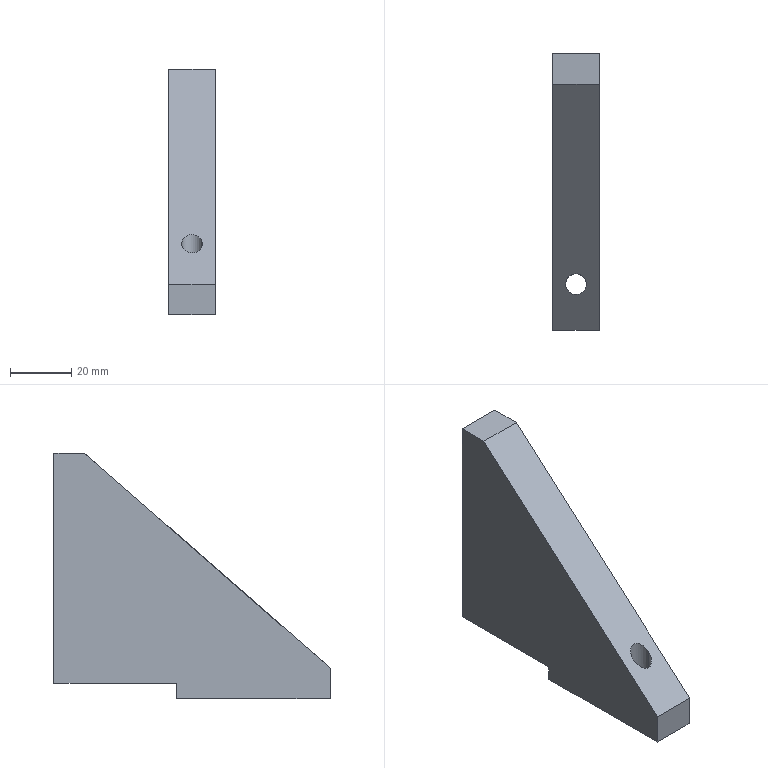Component | SolidWorks | FrameAssembly-1_SupportBlock-2 | 1 solid | 31 faces | box 15 x 90 x 80 mm | volume 59644 mm3 | cone 14 | plane 9 | cylinder 8 | commonest cylinder face diameters 6.8 x8
build123d program:
from build123d import *

# Parameters (mm, degrees)
BOSS_EXTRUDE1_DEPTH            = 15
SKETCH2_W                      = 5
SKETCH2_H                      = 40
CUT_EXTRUDE1_DEPTH             = 122.347
F_6_8_6_8_DIAMETER_HOLE1_D     = 6.8
F_6_8_6_8_DIAMETER_HOLE2_D     = 6.8
F_6_8_6_8_DIAMETER_HOLE2_DEPTH = 22.25
F_6_8_6_8_DIAMETER_HOLE2_TIP   = 2.043
F_6_8_6_8_DIAMETER_HOLE3_D     = 6.8
F_6_8_6_8_DIAMETER_HOLE3_DEPTH = 22.25
F_6_8_6_8_DIAMETER_HOLE3_TIP   = 2.043
CHAMFER1_SIZE                  = 0.625


with BuildPart() as part:
    # Sketch1 → Boss-Extrude1 (new body)
    with BuildSketch(Plane.XY.offset(7.5)):
        Polygon((80, 80), (80, 90), (0, 90), (0, 0), (10, 0), align=None)
    extrude(amount=-BOSS_EXTRUDE1_DEPTH)

    # Sketch2 → Cut-Extrude1 (cut, through all)
    with BuildSketch(Plane(origin=(0, 0, -7.5), x_dir=(-1, 0, 0), z_dir=(0, 0, -1))):
        with Locations((-2.5, 70)):
            Rectangle(SKETCH2_W, SKETCH2_H)
    extrude(amount=-CUT_EXTRUDE1_DEPTH, mode=Mode.SUBTRACT)

    # 6.8 _6.8_ Diameter Hole1 (through all)
    with Locations(Plane.ZY):
        with Locations((0, 15)):
            Hole(F_6_8_6_8_DIAMETER_HOLE1_D / 2)

    # 6.8 _6.8_ Diameter Hole2
    with Locations(Plane(origin=(0, 90, 0), x_dir=(1, 0, 0), z_dir=(0, 1, 0))):
        with Locations((60, 0), (20, 0)):
            Hole(F_6_8_6_8_DIAMETER_HOLE2_D / 2, depth=F_6_8_6_8_DIAMETER_HOLE2_DEPTH)
            with Locations((0, 0, -(F_6_8_6_8_DIAMETER_HOLE2_DEPTH + F_6_8_6_8_DIAMETER_HOLE2_TIP / 2))):  # 118° drill point
                Cone(0, F_6_8_6_8_DIAMETER_HOLE2_D / 2, F_6_8_6_8_DIAMETER_HOLE2_TIP, mode=Mode.SUBTRACT)

    # 6.8 _6.8_ Diameter Hole3
    with Locations(Plane.ZY):
        with Locations((0, 40)):
            Hole(F_6_8_6_8_DIAMETER_HOLE3_D / 2, depth=F_6_8_6_8_DIAMETER_HOLE3_DEPTH)
            with Locations((0, 0, -(F_6_8_6_8_DIAMETER_HOLE3_DEPTH + F_6_8_6_8_DIAMETER_HOLE3_TIP / 2))):  # 118° drill point
                Cone(0, F_6_8_6_8_DIAMETER_HOLE3_D / 2, F_6_8_6_8_DIAMETER_HOLE3_TIP, mode=Mode.SUBTRACT)

    # Chamfer1
    chamfer1_edges = [part.edges().sort_by_distance(p)[0] for p in [
        (0, 15, 3.4),
        (23.4, 90, 0),
        (63.4, 90, 0),
        (0, 40, 3.4),
    ]]
    chamfer(chamfer1_edges, length=CHAMFER1_SIZE)


solid = part.part

# Placed as in the assembly
solid = solid.moved(Location((-141.246, 270.373, -16.5), (0, -90, 0)))
STEP:
#1=COLOUR_RGB('',0.7922,0.8196,0.9333);
#2=FILL_AREA_STYLE_COLOUR('',#1);
#3=FILL_AREA_STYLE('',(#2));
#4=SURFACE_STYLE_FILL_AREA(#3);
#5=SURFACE_SIDE_STYLE('',(#4));
#6=SURFACE_STYLE_USAGE(.BOTH.,#5);
#7=PRESENTATION_STYLE_ASSIGNMENT((#6));
#8=CARTESIAN_POINT('',(-5.427,12.219,-0.625));
#9=VERTEX_POINT('',#8);
#10=CARTESIAN_POINT('',(-5.695,12.219,-0.625));
#11=VERTEX_POINT('',#10);
#12=CARTESIAN_POINT('',(-5.561,12.219,-0.625));
#13=DIRECTION('',(-0.,0.,-1.));
#14=DIRECTION('',(-1.,0.,0.));
#15=AXIS2_PLACEMENT_3D('',#12,#13,#14);
#16=CIRCLE('',#15,0.1339);
#17=EDGE_CURVE('',#9,#11,#16,.T.);
#18=ORIENTED_EDGE('',*,*,#17,.F.);
#19=CARTESIAN_POINT('',(-5.402,12.219,-0.6496));
#20=VERTEX_POINT('',#19);
#21=CARTESIAN_POINT('',(-5.427,12.219,-0.625));
#22=DIRECTION('',(0.7071,0.,-0.7071));
#23=VECTOR('',#22,39.37);
#24=LINE('',#21,#23);
#25=EDGE_CURVE('',#9,#20,#24,.T.);
#26=ORIENTED_EDGE('',*,*,#25,.T.);
#27=CARTESIAN_POINT('',(-5.719,12.219,-0.6496));
#28=VERTEX_POINT('',#27);
#29=CARTESIAN_POINT('',(-5.561,12.219,-0.6496));
#30=DIRECTION('',(-0.,0.,1.));
#31=DIRECTION('',(0.,-1.,0.));
#32=AXIS2_PLACEMENT_3D('',#29,#30,#31);
#33=CIRCLE('',#32,0.1585);
#34=EDGE_CURVE('',#28,#20,#33,.T.);
#35=ORIENTED_EDGE('',*,*,#34,.F.);
#36=CARTESIAN_POINT('',(-5.695,12.219,-0.625));
#37=DIRECTION('',(-0.7071,-0.,-0.7071));
#38=VECTOR('',#37,39.37);
#39=LINE('',#36,#38);
#40=EDGE_CURVE('',#11,#28,#39,.T.);
#41=ORIENTED_EDGE('',*,*,#40,.F.);
#42=EDGE_LOOP('',(#18,#26,#35,#41));
#43=FACE_OUTER_BOUND('',#42,.T.);
#44=CARTESIAN_POINT('',(-5.561,12.219,-0.625));
#45=DIRECTION('',(-0.,0.,-1.));
#46=DIRECTION('',(-1.,0.,0.));
#47=AXIS2_PLACEMENT_3D('',#44,#45,#46);
#48=CONICAL_SURFACE('',#47,0.1339,0.7854);
#49=ADVANCED_FACE('',(#43),#48,.F.);
#50=CARTESIAN_POINT('',(-5.427,11.235,-0.625));
#51=VERTEX_POINT('',#50);
#52=CARTESIAN_POINT('',(-5.695,11.235,-0.625));
#53=VERTEX_POINT('',#52);
#54=CARTESIAN_POINT('',(-5.561,11.235,-0.625));
#55=DIRECTION('',(-0.,0.,-1.));
#56=DIRECTION('',(-1.,0.,0.));
#57=AXIS2_PLACEMENT_3D('',#54,#55,#56);
#58=CIRCLE('',#57,0.1339);
#59=EDGE_CURVE('',#51,#53,#58,.T.);
#60=ORIENTED_EDGE('',*,*,#59,.F.);
#61=CARTESIAN_POINT('',(-5.402,11.235,-0.6496));
#62=VERTEX_POINT('',#61);
#63=CARTESIAN_POINT('',(-5.427,11.235,-0.625));
#64=DIRECTION('',(0.7071,0.,-0.7071));
#65=VECTOR('',#64,39.37);
#66=LINE('',#63,#65);
#67=EDGE_CURVE('',#51,#62,#66,.T.);
#68=ORIENTED_EDGE('',*,*,#67,.T.);
#69=CARTESIAN_POINT('',(-5.719,11.235,-0.6496));
#70=VERTEX_POINT('',#69);
#71=CARTESIAN_POINT('',(-5.561,11.235,-0.6496));
#72=DIRECTION('',(-0.,0.,1.));
#73=DIRECTION('',(0.,-1.,0.));
#74=AXIS2_PLACEMENT_3D('',#71,#72,#73);
#75=CIRCLE('',#74,0.1585);
#76=EDGE_CURVE('',#70,#62,#75,.T.);
#77=ORIENTED_EDGE('',*,*,#76,.F.);
#78=CARTESIAN_POINT('',(-5.695,11.235,-0.625));
#79=DIRECTION('',(-0.7071,0.,-0.7071));
#80=VECTOR('',#79,39.37);
#81=LINE('',#78,#80);
#82=EDGE_CURVE('',#53,#70,#81,.T.);
#83=ORIENTED_EDGE('',*,*,#82,.F.);
#84=EDGE_LOOP('',(#60,#68,#77,#83));
#85=FACE_OUTER_BOUND('',#84,.T.);
#86=CARTESIAN_POINT('',(-5.561,11.235,-0.625));
#87=DIRECTION('',(-0.,0.,-1.));
#88=DIRECTION('',(-1.,0.,0.));
#89=AXIS2_PLACEMENT_3D('',#86,#87,#88);
#90=CONICAL_SURFACE('',#89,0.1339,0.7854);
#91=ADVANCED_FACE('',(#85),#90,.F.);
#92=CARTESIAN_POINT('',(-5.427,14.163,1.713));
#93=VERTEX_POINT('',#92);
#94=CARTESIAN_POINT('',(-5.695,14.163,1.713));
#95=VERTEX_POINT('',#94);
#96=CARTESIAN_POINT('',(-5.561,14.163,1.713));
#97=DIRECTION('',(-0.,1.,0.));
#98=DIRECTION('',(-1.,0.,0.));
#99=AXIS2_PLACEMENT_3D('',#96,#97,#98);
#100=CIRCLE('',#99,0.1339);
#101=EDGE_CURVE('',#93,#95,#100,.T.);
#102=ORIENTED_EDGE('',*,*,#101,.F.);
#103=CARTESIAN_POINT('',(-5.402,14.188,1.713));
#104=VERTEX_POINT('',#103);
#105=CARTESIAN_POINT('',(-5.427,14.163,1.713));
#106=DIRECTION('',(0.7071,0.7071,0.));
#107=VECTOR('',#106,39.37);
#108=LINE('',#105,#107);
#109=EDGE_CURVE('',#93,#104,#108,.T.);
#110=ORIENTED_EDGE('',*,*,#109,.T.);
#111=CARTESIAN_POINT('',(-5.719,14.188,1.713));
#112=VERTEX_POINT('',#111);
#113=CARTESIAN_POINT('',(-5.561,14.188,1.713));
#114=DIRECTION('',(0.,-1.,0.));
#115=DIRECTION('',(0.,0.,-1.));
#116=AXIS2_PLACEMENT_3D('',#113,#114,#115);
#117=CIRCLE('',#116,0.1585);
#118=EDGE_CURVE('',#112,#104,#117,.T.);
#119=ORIENTED_EDGE('',*,*,#118,.F.);
#120=CARTESIAN_POINT('',(-5.695,14.163,1.713));
#121=DIRECTION('',(-0.7071,0.7071,0.));
#122=VECTOR('',#121,39.37);
#123=LINE('',#120,#122);
#124=EDGE_CURVE('',#95,#112,#123,.T.);
#125=ORIENTED_EDGE('',*,*,#124,.F.);
#126=EDGE_LOOP('',(#102,#110,#119,#125));
#127=FACE_OUTER_BOUND('',#126,.T.);
#128=CARTESIAN_POINT('',(-5.561,14.163,1.713));
#129=DIRECTION('',(-0.,1.,0.));
#130=DIRECTION('',(-1.,0.,0.));
#131=AXIS2_PLACEMENT_3D('',#128,#129,#130);
#132=CONICAL_SURFACE('',#131,0.1339,0.7854);
#133=ADVANCED_FACE('',(#127),#132,.F.);
#134=CARTESIAN_POINT('',(-5.427,14.163,0.1378));
#135=VERTEX_POINT('',#134);
#136=CARTESIAN_POINT('',(-5.695,14.163,0.1378));
#137=VERTEX_POINT('',#136);
#138=CARTESIAN_POINT('',(-5.561,14.163,0.1378));
#139=DIRECTION('',(-0.,1.,0.));
#140=DIRECTION('',(-1.,0.,0.));
#141=AXIS2_PLACEMENT_3D('',#138,#139,#140);
#142=CIRCLE('',#141,0.1339);
#143=EDGE_CURVE('',#135,#137,#142,.T.);
#144=ORIENTED_EDGE('',*,*,#143,.F.);
#145=CARTESIAN_POINT('',(-5.402,14.188,0.1378));
#146=VERTEX_POINT('',#145);
#147=CARTESIAN_POINT('',(-5.427,14.163,0.1378));
#148=DIRECTION('',(0.7071,0.7071,0.));
#149=VECTOR('',#148,39.37);
#150=LINE('',#147,#149);
#151=EDGE_CURVE('',#135,#146,#150,.T.);
#152=ORIENTED_EDGE('',*,*,#151,.T.);
#153=CARTESIAN_POINT('',(-5.719,14.188,0.1378));
#154=VERTEX_POINT('',#153);
#155=CARTESIAN_POINT('',(-5.561,14.188,0.1378));
#156=DIRECTION('',(0.,-1.,0.));
#157=DIRECTION('',(0.,0.,-1.));
#158=AXIS2_PLACEMENT_3D('',#155,#156,#157);
#159=CIRCLE('',#158,0.1585);
#160=EDGE_CURVE('',#154,#146,#159,.T.);
#161=ORIENTED_EDGE('',*,*,#160,.F.);
#162=CARTESIAN_POINT('',(-5.695,14.163,0.1378));
#163=DIRECTION('',(-0.7071,0.7071,0.));
#164=VECTOR('',#163,39.37);
#165=LINE('',#162,#164);
#166=EDGE_CURVE('',#137,#154,#165,.T.);
#167=ORIENTED_EDGE('',*,*,#166,.F.);
#168=EDGE_LOOP('',(#144,#152,#161,#167));
#169=FACE_OUTER_BOUND('',#168,.T.);
#170=CARTESIAN_POINT('',(-5.561,14.163,0.1378));
#171=DIRECTION('',(-0.,1.,0.));
#172=DIRECTION('',(-1.,0.,0.));
#173=AXIS2_PLACEMENT_3D('',#170,#171,#172);
#174=CONICAL_SURFACE('',#173,0.1339,0.7854);
#175=ADVANCED_FACE('',(#169),#174,.F.);
#176=CARTESIAN_POINT('',(-5.427,12.219,0.2264));
#177=VERTEX_POINT('',#176);
#178=CARTESIAN_POINT('',(-5.695,12.219,0.2264));
#179=VERTEX_POINT('',#178);
#180=CARTESIAN_POINT('',(-5.561,12.219,0.2264));
#181=DIRECTION('',(-0.,0.,-1.));
#182=DIRECTION('',(-1.,0.,0.));
#183=AXIS2_PLACEMENT_3D('',#180,#181,#182);
#184=CIRCLE('',#183,0.1339);
#185=EDGE_CURVE('',#177,#179,#184,.T.);
#186=ORIENTED_EDGE('',*,*,#185,.F.);
#187=CARTESIAN_POINT('',(-5.427,12.219,-0.6496));
#188=DIRECTION('',(-0.,0.,-1.));
#189=VECTOR('',#188,39.37);
#190=LINE('',#187,#189);
#191=EDGE_CURVE('',#177,#9,#190,.T.);
#192=ORIENTED_EDGE('',*,*,#191,.T.);
#193=ORIENTED_EDGE('',*,*,#17,.T.);
#194=CARTESIAN_POINT('',(-5.695,12.219,-0.6496));
#195=DIRECTION('',(-0.,0.,-1.));
#196=VECTOR('',#195,39.37);
#197=LINE('',#194,#196);
#198=EDGE_CURVE('',#179,#11,#197,.T.);
#199=ORIENTED_EDGE('',*,*,#198,.F.);
#200=EDGE_LOOP('',(#186,#192,#193,#199));
#201=FACE_OUTER_BOUND('',#200,.T.);
#202=CARTESIAN_POINT('',(-5.561,12.219,-0.6496));
#203=DIRECTION('',(-0.,0.,-1.));
#204=DIRECTION('',(-1.,0.,0.));
#205=AXIS2_PLACEMENT_3D('',#202,#203,#204);
#206=CYLINDRICAL_SURFACE('',#205,0.1339);
#207=ADVANCED_FACE('',(#201),#206,.F.);
#208=CARTESIAN_POINT('',(-5.561,12.219,0.3068));
#209=VERTEX_POINT('',#208);
#210=CARTESIAN_POINT('',(-5.695,12.219,0.2264));
#211=DIRECTION('',(-0.8572,-0.,-0.515));
#212=VECTOR('',#211,39.37);
#213=LINE('',#210,#212);
#214=EDGE_CURVE('',#209,#179,#213,.T.);
#215=ORIENTED_EDGE('',*,*,#214,.F.);
#216=CARTESIAN_POINT('',(-5.427,12.219,0.2264));
#217=DIRECTION('',(0.8572,0.,-0.515));
#218=VECTOR('',#217,39.37);
#219=LINE('',#216,#218);
#220=EDGE_CURVE('',#209,#177,#219,.T.);
#221=ORIENTED_EDGE('',*,*,#220,.T.);
#222=ORIENTED_EDGE('',*,*,#185,.T.);
#223=EDGE_LOOP('',(#215,#221,#222));
#224=FACE_OUTER_BOUND('',#223,.T.);
#225=CARTESIAN_POINT('',(-5.561,12.219,0.2264));
#226=DIRECTION('',(-0.,0.,-1.));
#227=DIRECTION('',(-1.,0.,0.));
#228=AXIS2_PLACEMENT_3D('',#225,#226,#227);
#229=CONICAL_SURFACE('',#228,0.1339,1.03);
#230=ADVANCED_FACE('',(#224),#229,.F.);
#231=CARTESIAN_POINT('',(-5.427,13.312,1.713));
#232=VERTEX_POINT('',#231);
#233=CARTESIAN_POINT('',(-5.695,13.312,1.713));
#234=VERTEX_POINT('',#233);
#235=CARTESIAN_POINT('',(-5.561,13.312,1.713));
#236=DIRECTION('',(-0.,1.,0.));
#237=DIRECTION('',(-1.,0.,0.));
#238=AXIS2_PLACEMENT_3D('',#235,#236,#237);
#239=CIRCLE('',#238,0.1339);
#240=EDGE_CURVE('',#232,#234,#239,.T.);
#241=ORIENTED_EDGE('',*,*,#240,.F.);
#242=CARTESIAN_POINT('',(-5.427,14.188,1.713));
#243=DIRECTION('',(-0.,1.,0.));
#244=VECTOR('',#243,39.37);
#245=LINE('',#242,#244);
#246=EDGE_CURVE('',#232,#93,#245,.T.);
#247=ORIENTED_EDGE('',*,*,#246,.T.);
#248=ORIENTED_EDGE('',*,*,#101,.T.);
#249=CARTESIAN_POINT('',(-5.695,14.188,1.713));
#250=DIRECTION('',(-0.,1.,0.));
#251=VECTOR('',#250,39.37);
#252=LINE('',#249,#251);
#253=EDGE_CURVE('',#234,#95,#252,.T.);
#254=ORIENTED_EDGE('',*,*,#253,.F.);
#255=EDGE_LOOP('',(#241,#247,#248,#254));
#256=FACE_OUTER_BOUND('',#255,.T.);
#257=CARTESIAN_POINT('',(-5.561,14.188,1.713));
#258=DIRECTION('',(-0.,1.,0.));
#259=DIRECTION('',(-1.,0.,0.));
#260=AXIS2_PLACEMENT_3D('',#257,#258,#259);
#261=CYLINDRICAL_SURFACE('',#260,0.1339);
#262=ADVANCED_FACE('',(#256),#261,.F.);
#263=CARTESIAN_POINT('',(-5.561,13.232,1.713));
#264=VERTEX_POINT('',#263);
#265=CARTESIAN_POINT('',(-5.695,13.312,1.713));
#266=DIRECTION('',(-0.8572,0.515,0.));
#267=VECTOR('',#266,39.37);
#268=LINE('',#265,#267);
#269=EDGE_CURVE('',#264,#234,#268,.T.);
#270=ORIENTED_EDGE('',*,*,#269,.F.);
#271=CARTESIAN_POINT('',(-5.427,13.312,1.713));
#272=DIRECTION('',(0.8572,0.515,0.));
#273=VECTOR('',#272,39.37);
#274=LINE('',#271,#273);
#275=EDGE_CURVE('',#264,#232,#274,.T.);
#276=ORIENTED_EDGE('',*,*,#275,.T.);
#277=ORIENTED_EDGE('',*,*,#240,.T.);
#278=EDGE_LOOP('',(#270,#276,#277));
#279=FACE_OUTER_BOUND('',#278,.T.);
#280=CARTESIAN_POINT('',(-5.561,13.312,1.713));
#281=DIRECTION('',(-0.,1.,0.));
#282=DIRECTION('',(-1.,0.,0.));
#283=AXIS2_PLACEMENT_3D('',#280,#281,#282);
#284=CONICAL_SURFACE('',#283,0.1339,1.03);
#285=ADVANCED_FACE('',(#279),#284,.F.);
#286=CARTESIAN_POINT('',(-5.427,13.312,0.1378));
#287=VERTEX_POINT('',#286);
#288=CARTESIAN_POINT('',(-5.695,13.312,0.1378));
#289=VERTEX_POINT('',#288);
#290=CARTESIAN_POINT('',(-5.561,13.312,0.1378));
#291=DIRECTION('',(-0.,1.,0.));
#292=DIRECTION('',(-1.,0.,0.));
#293=AXIS2_PLACEMENT_3D('',#290,#291,#292);
#294=CIRCLE('',#293,0.1339);
#295=EDGE_CURVE('',#287,#289,#294,.T.);
#296=ORIENTED_EDGE('',*,*,#295,.F.);
#297=CARTESIAN_POINT('',(-5.427,14.188,0.1378));
#298=DIRECTION('',(-0.,1.,0.));
#299=VECTOR('',#298,39.37);
#300=LINE('',#297,#299);
#301=EDGE_CURVE('',#287,#135,#300,.T.);
#302=ORIENTED_EDGE('',*,*,#301,.T.);
#303=ORIENTED_EDGE('',*,*,#143,.T.);
#304=CARTESIAN_POINT('',(-5.695,14.188,0.1378));
#305=DIRECTION('',(-0.,1.,0.));
#306=VECTOR('',#305,39.37);
#307=LINE('',#304,#306);
#308=EDGE_CURVE('',#289,#137,#307,.T.);
#309=ORIENTED_EDGE('',*,*,#308,.F.);
#310=EDGE_LOOP('',(#296,#302,#303,#309));
#311=FACE_OUTER_BOUND('',#310,.T.);
#312=CARTESIAN_POINT('',(-5.561,14.188,0.1378));
#313=DIRECTION('',(-0.,1.,0.));
#314=DIRECTION('',(-1.,0.,0.));
#315=AXIS2_PLACEMENT_3D('',#312,#313,#314);
#316=CYLINDRICAL_SURFACE('',#315,0.1339);
#317=ADVANCED_FACE('',(#311),#316,.F.);
#318=CARTESIAN_POINT('',(-5.561,13.232,0.1378));
#319=VERTEX_POINT('',#318);
#320=CARTESIAN_POINT('',(-5.695,13.312,0.1378));
#321=DIRECTION('',(-0.8572,0.515,0.));
#322=VECTOR('',#321,39.37);
#323=LINE('',#320,#322);
#324=EDGE_CURVE('',#319,#289,#323,.T.);
#325=ORIENTED_EDGE('',*,*,#324,.F.);
#326=CARTESIAN_POINT('',(-5.427,13.312,0.1378));
#327=DIRECTION('',(0.8572,0.515,0.));
#328=VECTOR('',#327,39.37);
#329=LINE('',#326,#328);
#330=EDGE_CURVE('',#319,#287,#329,.T.);
#331=ORIENTED_EDGE('',*,*,#330,.T.);
#332=ORIENTED_EDGE('',*,*,#295,.T.);
#333=EDGE_LOOP('',(#325,#331,#332));
#334=FACE_OUTER_BOUND('',#333,.T.);
#335=CARTESIAN_POINT('',(-5.561,13.312,0.1378));
#336=DIRECTION('',(-0.,1.,0.));
#337=DIRECTION('',(-1.,0.,0.));
#338=AXIS2_PLACEMENT_3D('',#335,#336,#337);
#339=CONICAL_SURFACE('',#338,0.1339,1.03);
#340=ADVANCED_FACE('',(#334),#339,.F.);
#341=CARTESIAN_POINT('',(-5.695,11.235,0.2608));
#342=VERTEX_POINT('',#341);
#343=CARTESIAN_POINT('',(-5.427,11.235,0.2608));
#344=VERTEX_POINT('',#343);
#345=CARTESIAN_POINT('',(-5.695,11.235,0.2608));
#346=CARTESIAN_POINT('',(-5.695,10.967,0.02657));
#347=CARTESIAN_POINT('',(-5.427,10.967,0.02657));
#348=CARTESIAN_POINT('',(-5.427,11.235,0.2608));
#349=(BOUNDED_CURVE()B_SPLINE_CURVE(3,(#345,#346,#347,#348),.UNSPECIFIED.,.F.,.F.)B_SPLINE_CURVE_WITH_KNOTS((4,4),(4.712,7.854),.UNSPECIFIED.)CURVE()GEOMETRIC_REPRESENTATION_ITEM()RATIONAL_B_SPLINE_CURVE((1.,0.3333,0.3333,1.))REPRESENTATION_ITEM(''));
#350=EDGE_CURVE('',#342,#344,#349,.T.);
#351=ORIENTED_EDGE('',*,*,#350,.T.);
#352=CARTESIAN_POINT('',(-5.427,11.235,-0.6496));
#353=DIRECTION('',(-0.,0.,-1.));
#354=VECTOR('',#353,39.37);
#355=LINE('',#352,#354);
#356=EDGE_CURVE('',#344,#51,#355,.T.);
#357=ORIENTED_EDGE('',*,*,#356,.T.);
#358=ORIENTED_EDGE('',*,*,#59,.T.);
#359=CARTESIAN_POINT('',(-5.695,11.235,-0.6496));
#360=DIRECTION('',(-0.,0.,-1.));
#361=VECTOR('',#360,39.37);
#362=LINE('',#359,#361);
#363=EDGE_CURVE('',#342,#53,#362,.T.);
#364=ORIENTED_EDGE('',*,*,#363,.F.);
#365=EDGE_LOOP('',(#351,#357,#358,#364));
#366=FACE_OUTER_BOUND('',#365,.T.);
#367=CARTESIAN_POINT('',(-5.561,11.235,-0.6496));
#368=DIRECTION('',(-0.,0.,-1.));
#369=DIRECTION('',(-1.,0.,0.));
#370=AXIS2_PLACEMENT_3D('',#367,#368,#369);
#371=CYLINDRICAL_SURFACE('',#370,0.1339);
#372=ADVANCED_FACE('',(#366),#371,.F.);
#373=ORIENTED_EDGE('',*,*,#350,.F.);
#374=CARTESIAN_POINT('',(-5.427,11.235,0.2608));
#375=CARTESIAN_POINT('',(-5.427,11.503,0.4951));
#376=CARTESIAN_POINT('',(-5.695,11.503,0.4951));
#377=CARTESIAN_POINT('',(-5.695,11.235,0.2608));
#378=(BOUNDED_CURVE()B_SPLINE_CURVE(3,(#374,#375,#376,#377),.UNSPECIFIED.,.F.,.F.)B_SPLINE_CURVE_WITH_KNOTS((4,4),(1.571,4.712),.UNSPECIFIED.)CURVE()GEOMETRIC_REPRESENTATION_ITEM()RATIONAL_B_SPLINE_CURVE((1.,0.3333,0.3333,1.))REPRESENTATION_ITEM(''));
#379=EDGE_CURVE('',#344,#342,#378,.T.);
#380=ORIENTED_EDGE('',*,*,#379,.F.);
#381=EDGE_LOOP('',(#373,#380));
#382=FACE_BOUND('',#381,.T.);
#383=CARTESIAN_POINT('',(-5.856,10.645,-0.2559));
#384=VERTEX_POINT('',#383);
#385=CARTESIAN_POINT('',(-5.856,13.794,2.5));
#386=VERTEX_POINT('',#385);
#387=CARTESIAN_POINT('',(-5.856,10.645,-0.2559));
#388=DIRECTION('',(-0.,0.7526,0.6585));
#389=VECTOR('',#388,39.37);
#390=LINE('',#387,#389);
#391=EDGE_CURVE('',#384,#386,#390,.T.);
#392=ORIENTED_EDGE('',*,*,#391,.F.);
#393=CARTESIAN_POINT('',(-5.266,10.645,-0.2559));
#394=VERTEX_POINT('',#393);
#395=CARTESIAN_POINT('',(-5.266,10.645,-0.2559));
#396=DIRECTION('',(-1.,-0.,0.));
#397=VECTOR('',#396,39.37);
#398=LINE('',#395,#397);
#399=EDGE_CURVE('',#394,#384,#398,.T.);
#400=ORIENTED_EDGE('',*,*,#399,.F.);
#401=CARTESIAN_POINT('',(-5.266,13.794,2.5));
#402=VERTEX_POINT('',#401);
#403=CARTESIAN_POINT('',(-5.266,10.645,-0.2559));
#404=DIRECTION('',(-0.,0.7526,0.6585));
#405=VECTOR('',#404,39.37);
#406=LINE('',#403,#405);
#407=EDGE_CURVE('',#394,#402,#406,.T.);
#408=ORIENTED_EDGE('',*,*,#407,.T.);
#409=CARTESIAN_POINT('',(-5.266,13.794,2.5));
#410=DIRECTION('',(-1.,-0.,0.));
#411=VECTOR('',#410,39.37);
#412=LINE('',#409,#411);
#413=EDGE_CURVE('',#402,#386,#412,.T.);
#414=ORIENTED_EDGE('',*,*,#413,.T.);
#415=EDGE_LOOP('',(#392,#400,#408,#414));
#416=FACE_OUTER_BOUND('',#415,.T.);
#417=CARTESIAN_POINT('',(-5.266,10.645,-0.2559));
#418=DIRECTION('',(0.,-0.6585,0.7526));
#419=DIRECTION('',(-0.,0.7526,0.6585));
#420=AXIS2_PLACEMENT_3D('',#417,#418,#419);
#421=PLANE('',#420);
#422=ADVANCED_FACE('',(#382,#416),#421,.T.);
#423=CARTESIAN_POINT('',(-5.856,10.645,-0.6496));
#424=VERTEX_POINT('',#423);
#425=CARTESIAN_POINT('',(-5.856,10.645,-0.6496));
#426=DIRECTION('',(-0.,0.,1.));
#427=VECTOR('',#426,39.37);
#428=LINE('',#425,#427);
#429=EDGE_CURVE('',#424,#384,#428,.T.);
#430=ORIENTED_EDGE('',*,*,#429,.F.);
#431=CARTESIAN_POINT('',(-5.266,10.645,-0.6496));
#432=VERTEX_POINT('',#431);
#433=CARTESIAN_POINT('',(-5.266,10.645,-0.6496));
#434=DIRECTION('',(-1.,-0.,0.));
#435=VECTOR('',#434,39.37);
#436=LINE('',#433,#435);
#437=EDGE_CURVE('',#432,#424,#436,.T.);
#438=ORIENTED_EDGE('',*,*,#437,.F.);
#439=CARTESIAN_POINT('',(-5.266,10.645,-0.6496));
#440=DIRECTION('',(-0.,0.,1.));
#441=VECTOR('',#440,39.37);
#442=LINE('',#439,#441);
#443=EDGE_CURVE('',#432,#394,#442,.T.);
#444=ORIENTED_EDGE('',*,*,#443,.T.);
#445=ORIENTED_EDGE('',*,*,#399,.T.);
#446=EDGE_LOOP('',(#430,#438,#444,#445));
#447=FACE_OUTER_BOUND('',#446,.T.);
#448=CARTESIAN_POINT('',(-5.266,10.645,-0.6496));
#449=DIRECTION('',(0.,-1.,0.));
#450=DIRECTION('',(-0.,0.,1.));
#451=AXIS2_PLACEMENT_3D('',#448,#449,#450);
#452=PLANE('',#451);
#453=ADVANCED_FACE('',(#447),#452,.T.);
#454=ORIENTED_EDGE('',*,*,#76,.T.);
#455=CARTESIAN_POINT('',(-5.561,11.235,-0.6496));
#456=DIRECTION('',(-0.,0.,1.));
#457=DIRECTION('',(0.,-1.,0.));
#458=AXIS2_PLACEMENT_3D('',#455,#456,#457);
#459=CIRCLE('',#458,0.1585);
#460=EDGE_CURVE('',#62,#70,#459,.T.);
#461=ORIENTED_EDGE('',*,*,#460,.T.);
#462=EDGE_LOOP('',(#454,#461));
#463=FACE_BOUND('',#462,.T.);
#464=ORIENTED_EDGE('',*,*,#34,.T.);
#465=CARTESIAN_POINT('',(-5.561,12.219,-0.6496));
#466=DIRECTION('',(-0.,0.,1.));
#467=DIRECTION('',(0.,-1.,0.));
#468=AXIS2_PLACEMENT_3D('',#465,#466,#467);
#469=CIRCLE('',#468,0.1585);
#470=EDGE_CURVE('',#20,#28,#469,.T.);
#471=ORIENTED_EDGE('',*,*,#470,.T.);
#472=EDGE_LOOP('',(#464,#471));
#473=FACE_BOUND('',#472,.T.);
#474=CARTESIAN_POINT('',(-5.856,12.613,-0.6496));
#475=VERTEX_POINT('',#474);
#476=CARTESIAN_POINT('',(-5.266,12.613,-0.6496));
#477=VERTEX_POINT('',#476);
#478=CARTESIAN_POINT('',(-5.856,12.613,-0.6496));
#479=DIRECTION('',(1.,0.,-0.));
#480=VECTOR('',#479,39.37);
#481=LINE('',#478,#480);
#482=EDGE_CURVE('',#475,#477,#481,.T.);
#483=ORIENTED_EDGE('',*,*,#482,.T.);
#484=CARTESIAN_POINT('',(-5.266,14.188,-0.6496));
#485=DIRECTION('',(0.,-1.,0.));
#486=VECTOR('',#485,39.37);
#487=LINE('',#484,#486);
#488=EDGE_CURVE('',#477,#432,#487,.T.);
#489=ORIENTED_EDGE('',*,*,#488,.T.);
#490=ORIENTED_EDGE('',*,*,#437,.T.);
#491=CARTESIAN_POINT('',(-5.856,14.188,-0.6496));
#492=DIRECTION('',(0.,-1.,0.));
#493=VECTOR('',#492,39.37);
#494=LINE('',#491,#493);
#495=EDGE_CURVE('',#475,#424,#494,.T.);
#496=ORIENTED_EDGE('',*,*,#495,.F.);
#497=EDGE_LOOP('',(#483,#489,#490,#496));
#498=FACE_OUTER_BOUND('',#497,.T.);
#499=CARTESIAN_POINT('',(-5.266,14.188,-0.6496));
#500=DIRECTION('',(0.,-0.,-1.));
#501=DIRECTION('',(0.,-1.,0.));
#502=AXIS2_PLACEMENT_3D('',#499,#500,#501);
#503=PLANE('',#502);
#504=ADVANCED_FACE('',(#463,#473,#498),#503,.T.);
#505=ORIENTED_EDGE('',*,*,#160,.T.);
#506=CARTESIAN_POINT('',(-5.561,14.188,0.1378));
#507=DIRECTION('',(0.,-1.,0.));
#508=DIRECTION('',(0.,0.,-1.));
#509=AXIS2_PLACEMENT_3D('',#506,#507,#508);
#510=CIRCLE('',#509,0.1585);
#511=EDGE_CURVE('',#146,#154,#510,.T.);
#512=ORIENTED_EDGE('',*,*,#511,.T.);
#513=EDGE_LOOP('',(#505,#512));
#514=FACE_BOUND('',#513,.T.);
#515=ORIENTED_EDGE('',*,*,#118,.T.);
#516=CARTESIAN_POINT('',(-5.561,14.188,1.713));
#517=DIRECTION('',(0.,-1.,0.));
#518=DIRECTION('',(0.,0.,-1.));
#519=AXIS2_PLACEMENT_3D('',#516,#517,#518);
#520=CIRCLE('',#519,0.1585);
#521=EDGE_CURVE('',#104,#112,#520,.T.);
#522=ORIENTED_EDGE('',*,*,#521,.T.);
#523=EDGE_LOOP('',(#515,#522));
#524=FACE_BOUND('',#523,.T.);
#525=CARTESIAN_POINT('',(-5.856,14.188,-0.4528));
#526=VERTEX_POINT('',#525);
#527=CARTESIAN_POINT('',(-5.266,14.188,-0.4528));
#528=VERTEX_POINT('',#527);
#529=CARTESIAN_POINT('',(-5.856,14.188,-0.4528));
#530=DIRECTION('',(1.,0.,-0.));
#531=VECTOR('',#530,39.37);
#532=LINE('',#529,#531);
#533=EDGE_CURVE('',#526,#528,#532,.T.);
#534=ORIENTED_EDGE('',*,*,#533,.F.);
#535=CARTESIAN_POINT('',(-5.856,14.188,2.5));
#536=VERTEX_POINT('',#535);
#537=CARTESIAN_POINT('',(-5.856,14.188,2.5));
#538=DIRECTION('',(0.,-0.,-1.));
#539=VECTOR('',#538,39.37);
#540=LINE('',#537,#539);
#541=EDGE_CURVE('',#536,#526,#540,.T.);
#542=ORIENTED_EDGE('',*,*,#541,.F.);
#543=CARTESIAN_POINT('',(-5.266,14.188,2.5));
#544=VERTEX_POINT('',#543);
#545=CARTESIAN_POINT('',(-5.266,14.188,2.5));
#546=DIRECTION('',(-1.,-0.,0.));
#547=VECTOR('',#546,39.37);
#548=LINE('',#545,#547);
#549=EDGE_CURVE('',#544,#536,#548,.T.);
#550=ORIENTED_EDGE('',*,*,#549,.F.);
#551=CARTESIAN_POINT('',(-5.266,14.188,2.5));
#552=DIRECTION('',(0.,-0.,-1.));
#553=VECTOR('',#552,39.37);
#554=LINE('',#551,#553);
#555=EDGE_CURVE('',#544,#528,#554,.T.);
#556=ORIENTED_EDGE('',*,*,#555,.T.);
#557=EDGE_LOOP('',(#534,#542,#550,#556));
#558=FACE_OUTER_BOUND('',#557,.T.);
#559=CARTESIAN_POINT('',(-5.266,14.188,2.5));
#560=DIRECTION('',(-0.,1.,-0.));
#561=DIRECTION('',(0.,-0.,-1.));
#562=AXIS2_PLACEMENT_3D('',#559,#560,#561);
#563=PLANE('',#562);
#564=ADVANCED_FACE('',(#514,#524,#558),#563,.T.);
#565=CARTESIAN_POINT('',(-5.856,13.794,2.5));
#566=DIRECTION('',(-0.,1.,0.));
#567=VECTOR('',#566,39.37);
#568=LINE('',#565,#567);
#569=EDGE_CURVE('',#386,#536,#568,.T.);
#570=ORIENTED_EDGE('',*,*,#569,.F.);
#571=ORIENTED_EDGE('',*,*,#413,.F.);
#572=CARTESIAN_POINT('',(-5.266,13.794,2.5));
#573=DIRECTION('',(-0.,1.,0.));
#574=VECTOR('',#573,39.37);
#575=LINE('',#572,#574);
#576=EDGE_CURVE('',#402,#544,#575,.T.);
#577=ORIENTED_EDGE('',*,*,#576,.T.);
#578=ORIENTED_EDGE('',*,*,#549,.T.);
#579=EDGE_LOOP('',(#570,#571,#577,#578));
#580=FACE_OUTER_BOUND('',#579,.T.);
#581=CARTESIAN_POINT('',(-5.266,13.794,2.5));
#582=DIRECTION('',(0.,-0.,1.));
#583=DIRECTION('',(1.,0.,-0.));
#584=AXIS2_PLACEMENT_3D('',#581,#582,#583);
#585=PLANE('',#584);
#586=ADVANCED_FACE('',(#580),#585,.T.);
#587=ORIENTED_EDGE('',*,*,#488,.F.);
#588=CARTESIAN_POINT('',(-5.266,12.613,-0.4528));
#589=VERTEX_POINT('',#588);
#590=CARTESIAN_POINT('',(-5.266,12.613,-0.4528));
#591=DIRECTION('',(-0.,0.,-1.));
#592=VECTOR('',#591,39.37);
#593=LINE('',#590,#592);
#594=EDGE_CURVE('',#589,#477,#593,.T.);
#595=ORIENTED_EDGE('',*,*,#594,.F.);
#596=CARTESIAN_POINT('',(-5.266,14.188,-0.4528));
#597=DIRECTION('',(0.,-1.,-0.));
#598=VECTOR('',#597,39.37);
#599=LINE('',#596,#598);
#600=EDGE_CURVE('',#528,#589,#599,.T.);
#601=ORIENTED_EDGE('',*,*,#600,.F.);
#602=ORIENTED_EDGE('',*,*,#555,.F.);
#603=ORIENTED_EDGE('',*,*,#576,.F.);
#604=ORIENTED_EDGE('',*,*,#407,.F.);
#605=ORIENTED_EDGE('',*,*,#443,.F.);
#606=EDGE_LOOP('',(#587,#595,#601,#602,#603,#604,#605));
#607=FACE_OUTER_BOUND('',#606,.T.);
#608=CARTESIAN_POINT('',(-5.266,10.645,-0.6496));
#609=DIRECTION('',(-1.,-0.,0.));
#610=DIRECTION('',(0.,-0.,1.));
#611=AXIS2_PLACEMENT_3D('',#608,#609,#610);
#612=PLANE('',#611);
#613=ADVANCED_FACE('',(#607),#612,.F.);
#614=CARTESIAN_POINT('',(-5.856,12.613,-0.4528));
#615=VERTEX_POINT('',#614);
#616=CARTESIAN_POINT('',(-5.856,12.613,-0.4528));
#617=DIRECTION('',(-0.,0.,-1.));
#618=VECTOR('',#617,39.37);
#619=LINE('',#616,#618);
#620=EDGE_CURVE('',#615,#475,#619,.T.);
#621=ORIENTED_EDGE('',*,*,#620,.T.);
#622=ORIENTED_EDGE('',*,*,#495,.T.);
#623=ORIENTED_EDGE('',*,*,#429,.T.);
#624=ORIENTED_EDGE('',*,*,#391,.T.);
#625=ORIENTED_EDGE('',*,*,#569,.T.);
#626=ORIENTED_EDGE('',*,*,#541,.T.);
#627=CARTESIAN_POINT('',(-5.856,14.188,-0.4528));
#628=DIRECTION('',(0.,-1.,-0.));
#629=VECTOR('',#628,39.37);
#630=LINE('',#627,#629);
#631=EDGE_CURVE('',#526,#615,#630,.T.);
#632=ORIENTED_EDGE('',*,*,#631,.T.);
#633=EDGE_LOOP('',(#621,#622,#623,#624,#625,#626,#632));
#634=FACE_OUTER_BOUND('',#633,.T.);
#635=CARTESIAN_POINT('',(-5.856,10.645,-0.6496));
#636=DIRECTION('',(-1.,-0.,0.));
#637=DIRECTION('',(0.,-0.,1.));
#638=AXIS2_PLACEMENT_3D('',#635,#636,#637);
#639=PLANE('',#638);
#640=ADVANCED_FACE('',(#634),#639,.T.);
#641=ORIENTED_EDGE('',*,*,#594,.T.);
#642=ORIENTED_EDGE('',*,*,#482,.F.);
#643=ORIENTED_EDGE('',*,*,#620,.F.);
#644=CARTESIAN_POINT('',(-5.856,12.613,-0.4528));
#645=DIRECTION('',(1.,0.,-0.));
#646=VECTOR('',#645,39.37);
#647=LINE('',#644,#646);
#648=EDGE_CURVE('',#615,#589,#647,.T.);
#649=ORIENTED_EDGE('',*,*,#648,.T.);
#650=EDGE_LOOP('',(#641,#642,#643,#649));
#651=FACE_OUTER_BOUND('',#650,.T.);
#652=CARTESIAN_POINT('',(-5.856,12.613,-0.4528));
#653=DIRECTION('',(0.,-1.,-0.));
#654=DIRECTION('',(1.,0.,-0.));
#655=AXIS2_PLACEMENT_3D('',#652,#653,#654);
#656=PLANE('',#655);
#657=ADVANCED_FACE('',(#651),#656,.F.);
#658=ORIENTED_EDGE('',*,*,#600,.T.);
#659=ORIENTED_EDGE('',*,*,#648,.F.);
#660=ORIENTED_EDGE('',*,*,#631,.F.);
#661=ORIENTED_EDGE('',*,*,#533,.T.);
#662=EDGE_LOOP('',(#658,#659,#660,#661));
#663=FACE_OUTER_BOUND('',#662,.T.);
#664=CARTESIAN_POINT('',(-5.856,14.188,-0.4528));
#665=DIRECTION('',(0.,-0.,1.));
#666=DIRECTION('',(1.,0.,-0.));
#667=AXIS2_PLACEMENT_3D('',#664,#665,#666);
#668=PLANE('',#667);
#669=ADVANCED_FACE('',(#663),#668,.F.);
#670=ORIENTED_EDGE('',*,*,#356,.F.);
#671=ORIENTED_EDGE('',*,*,#379,.T.);
#672=ORIENTED_EDGE('',*,*,#363,.T.);
#673=CARTESIAN_POINT('',(-5.561,11.235,-0.625));
#674=DIRECTION('',(-0.,0.,-1.));
#675=DIRECTION('',(-1.,0.,0.));
#676=AXIS2_PLACEMENT_3D('',#673,#674,#675);
#677=CIRCLE('',#676,0.1339);
#678=EDGE_CURVE('',#53,#51,#677,.T.);
#679=ORIENTED_EDGE('',*,*,#678,.T.);
#680=EDGE_LOOP('',(#670,#671,#672,#679));
#681=FACE_OUTER_BOUND('',#680,.T.);
#682=CARTESIAN_POINT('',(-5.561,11.235,-0.6496));
#683=DIRECTION('',(-0.,0.,-1.));
#684=DIRECTION('',(-1.,0.,0.));
#685=AXIS2_PLACEMENT_3D('',#682,#683,#684);
#686=CYLINDRICAL_SURFACE('',#685,0.1339);
#687=ADVANCED_FACE('',(#681),#686,.F.);
#688=ORIENTED_EDGE('',*,*,#330,.F.);
#689=ORIENTED_EDGE('',*,*,#324,.T.);
#690=CARTESIAN_POINT('',(-5.561,13.312,0.1378));
#691=DIRECTION('',(-0.,1.,0.));
#692=DIRECTION('',(-1.,0.,0.));
#693=AXIS2_PLACEMENT_3D('',#690,#691,#692);
#694=CIRCLE('',#693,0.1339);
#695=EDGE_CURVE('',#289,#287,#694,.T.);
#696=ORIENTED_EDGE('',*,*,#695,.T.);
#697=EDGE_LOOP('',(#688,#689,#696));
#698=FACE_OUTER_BOUND('',#697,.T.);
#699=CARTESIAN_POINT('',(-5.561,13.312,0.1378));
#700=DIRECTION('',(-0.,1.,0.));
#701=DIRECTION('',(-1.,0.,0.));
#702=AXIS2_PLACEMENT_3D('',#699,#700,#701);
#703=CONICAL_SURFACE('',#702,0.1339,1.03);
#704=ADVANCED_FACE('',(#698),#703,.F.);
#705=ORIENTED_EDGE('',*,*,#301,.F.);
#706=ORIENTED_EDGE('',*,*,#695,.F.);
#707=ORIENTED_EDGE('',*,*,#308,.T.);
#708=CARTESIAN_POINT('',(-5.561,14.163,0.1378));
#709=DIRECTION('',(-0.,1.,0.));
#710=DIRECTION('',(-1.,0.,0.));
#711=AXIS2_PLACEMENT_3D('',#708,#709,#710);
#712=CIRCLE('',#711,0.1339);
#713=EDGE_CURVE('',#137,#135,#712,.T.);
#714=ORIENTED_EDGE('',*,*,#713,.T.);
#715=EDGE_LOOP('',(#705,#706,#707,#714));
#716=FACE_OUTER_BOUND('',#715,.T.);
#717=CARTESIAN_POINT('',(-5.561,14.188,0.1378));
#718=DIRECTION('',(-0.,1.,0.));
#719=DIRECTION('',(-1.,0.,0.));
#720=AXIS2_PLACEMENT_3D('',#717,#718,#719);
#721=CYLINDRICAL_SURFACE('',#720,0.1339);
#722=ADVANCED_FACE('',(#716),#721,.F.);
#723=ORIENTED_EDGE('',*,*,#275,.F.);
#724=ORIENTED_EDGE('',*,*,#269,.T.);
#725=CARTESIAN_POINT('',(-5.561,13.312,1.713));
#726=DIRECTION('',(-0.,1.,0.));
#727=DIRECTION('',(-1.,0.,0.));
#728=AXIS2_PLACEMENT_3D('',#725,#726,#727);
#729=CIRCLE('',#728,0.1339);
#730=EDGE_CURVE('',#234,#232,#729,.T.);
#731=ORIENTED_EDGE('',*,*,#730,.T.);
#732=EDGE_LOOP('',(#723,#724,#731));
#733=FACE_OUTER_BOUND('',#732,.T.);
#734=CARTESIAN_POINT('',(-5.561,13.312,1.713));
#735=DIRECTION('',(-0.,1.,0.));
#736=DIRECTION('',(-1.,0.,0.));
#737=AXIS2_PLACEMENT_3D('',#734,#735,#736);
#738=CONICAL_SURFACE('',#737,0.1339,1.03);
#739=ADVANCED_FACE('',(#733),#738,.F.);
#740=ORIENTED_EDGE('',*,*,#246,.F.);
#741=ORIENTED_EDGE('',*,*,#730,.F.);
#742=ORIENTED_EDGE('',*,*,#253,.T.);
#743=CARTESIAN_POINT('',(-5.561,14.163,1.713));
#744=DIRECTION('',(-0.,1.,0.));
#745=DIRECTION('',(-1.,0.,0.));
#746=AXIS2_PLACEMENT_3D('',#743,#744,#745);
#747=CIRCLE('',#746,0.1339);
#748=EDGE_CURVE('',#95,#93,#747,.T.);
#749=ORIENTED_EDGE('',*,*,#748,.T.);
#750=EDGE_LOOP('',(#740,#741,#742,#749));
#751=FACE_OUTER_BOUND('',#750,.T.);
#752=CARTESIAN_POINT('',(-5.561,14.188,1.713));
#753=DIRECTION('',(-0.,1.,0.));
#754=DIRECTION('',(-1.,0.,0.));
#755=AXIS2_PLACEMENT_3D('',#752,#753,#754);
#756=CYLINDRICAL_SURFACE('',#755,0.1339);
#757=ADVANCED_FACE('',(#751),#756,.F.);
#758=ORIENTED_EDGE('',*,*,#220,.F.);
#759=ORIENTED_EDGE('',*,*,#214,.T.);
#760=CARTESIAN_POINT('',(-5.561,12.219,0.2264));
#761=DIRECTION('',(-0.,0.,-1.));
#762=DIRECTION('',(-1.,0.,0.));
#763=AXIS2_PLACEMENT_3D('',#760,#761,#762);
#764=CIRCLE('',#763,0.1339);
#765=EDGE_CURVE('',#179,#177,#764,.T.);
#766=ORIENTED_EDGE('',*,*,#765,.T.);
#767=EDGE_LOOP('',(#758,#759,#766));
#768=FACE_OUTER_BOUND('',#767,.T.);
#769=CARTESIAN_POINT('',(-5.561,12.219,0.2264));
#770=DIRECTION('',(-0.,0.,-1.));
#771=DIRECTION('',(-1.,0.,0.));
#772=AXIS2_PLACEMENT_3D('',#769,#770,#771);
#773=CONICAL_SURFACE('',#772,0.1339,1.03);
#774=ADVANCED_FACE('',(#768),#773,.F.);
#775=ORIENTED_EDGE('',*,*,#191,.F.);
#776=ORIENTED_EDGE('',*,*,#765,.F.);
#777=ORIENTED_EDGE('',*,*,#198,.T.);
#778=CARTESIAN_POINT('',(-5.561,12.219,-0.625));
#779=DIRECTION('',(-0.,0.,-1.));
#780=DIRECTION('',(-1.,0.,0.));
#781=AXIS2_PLACEMENT_3D('',#778,#779,#780);
#782=CIRCLE('',#781,0.1339);
#783=EDGE_CURVE('',#11,#9,#782,.T.);
#784=ORIENTED_EDGE('',*,*,#783,.T.);
#785=EDGE_LOOP('',(#775,#776,#777,#784));
#786=FACE_OUTER_BOUND('',#785,.T.);
#787=CARTESIAN_POINT('',(-5.561,12.219,-0.6496));
#788=DIRECTION('',(-0.,0.,-1.));
#789=DIRECTION('',(-1.,0.,0.));
#790=AXIS2_PLACEMENT_3D('',#787,#788,#789);
#791=CYLINDRICAL_SURFACE('',#790,0.1339);
#792=ADVANCED_FACE('',(#786),#791,.F.);
#793=ORIENTED_EDGE('',*,*,#151,.F.);
#794=ORIENTED_EDGE('',*,*,#713,.F.);
#795=ORIENTED_EDGE('',*,*,#166,.T.);
#796=ORIENTED_EDGE('',*,*,#511,.F.);
#797=EDGE_LOOP('',(#793,#794,#795,#796));
#798=FACE_OUTER_BOUND('',#797,.T.);
#799=CARTESIAN_POINT('',(-5.561,14.163,0.1378));
#800=DIRECTION('',(-0.,1.,0.));
#801=DIRECTION('',(-1.,0.,0.));
#802=AXIS2_PLACEMENT_3D('',#799,#800,#801);
#803=CONICAL_SURFACE('',#802,0.1339,0.7854);
#804=ADVANCED_FACE('',(#798),#803,.F.);
#805=ORIENTED_EDGE('',*,*,#109,.F.);
#806=ORIENTED_EDGE('',*,*,#748,.F.);
#807=ORIENTED_EDGE('',*,*,#124,.T.);
#808=ORIENTED_EDGE('',*,*,#521,.F.);
#809=EDGE_LOOP('',(#805,#806,#807,#808));
#810=FACE_OUTER_BOUND('',#809,.T.);
#811=CARTESIAN_POINT('',(-5.561,14.163,1.713));
#812=DIRECTION('',(-0.,1.,0.));
#813=DIRECTION('',(-1.,0.,0.));
#814=AXIS2_PLACEMENT_3D('',#811,#812,#813);
#815=CONICAL_SURFACE('',#814,0.1339,0.7854);
#816=ADVANCED_FACE('',(#810),#815,.F.);
#817=ORIENTED_EDGE('',*,*,#67,.F.);
#818=ORIENTED_EDGE('',*,*,#678,.F.);
#819=ORIENTED_EDGE('',*,*,#82,.T.);
#820=ORIENTED_EDGE('',*,*,#460,.F.);
#821=EDGE_LOOP('',(#817,#818,#819,#820));
#822=FACE_OUTER_BOUND('',#821,.T.);
#823=CARTESIAN_POINT('',(-5.561,11.235,-0.625));
#824=DIRECTION('',(-0.,0.,-1.));
#825=DIRECTION('',(-1.,0.,0.));
#826=AXIS2_PLACEMENT_3D('',#823,#824,#825);
#827=CONICAL_SURFACE('',#826,0.1339,0.7854);
#828=ADVANCED_FACE('',(#822),#827,.F.);
#829=ORIENTED_EDGE('',*,*,#25,.F.);
#830=ORIENTED_EDGE('',*,*,#783,.F.);
#831=ORIENTED_EDGE('',*,*,#40,.T.);
#832=ORIENTED_EDGE('',*,*,#470,.F.);
#833=EDGE_LOOP('',(#829,#830,#831,#832));
#834=FACE_OUTER_BOUND('',#833,.T.);
#835=CARTESIAN_POINT('',(-5.561,12.219,-0.625));
#836=DIRECTION('',(-0.,0.,-1.));
#837=DIRECTION('',(-1.,0.,0.));
#838=AXIS2_PLACEMENT_3D('',#835,#836,#837);
#839=CONICAL_SURFACE('',#838,0.1339,0.7854);
#840=ADVANCED_FACE('',(#834),#839,.F.);
#841=CLOSED_SHELL('',(#49,#91,#133,#175,#207,#230,#262,#285,#317,#340,#372,#422,#453,#504,#564,#586,#613,#640,#657,#669,#687,#704,#722,#739,#757,#774,#792,#804,#816,#828,#840));
#842=MANIFOLD_SOLID_BREP('',#841);
#843=STYLED_ITEM('',(#7),#842);
#844=PRESENTATION_LAYER_ASSIGNMENT('','',(#843));
#845=CARTESIAN_POINT('',(0.,0.,0.));
#846=DIRECTION('',(0.,0.,1.));
#847=DIRECTION('',(1.,0.,0.));
#848=AXIS2_PLACEMENT_3D('',#845,#846,#847);
#849=(LENGTH_UNIT()NAMED_UNIT(*)SI_UNIT($,.METRE.));
#850=LENGTH_MEASURE_WITH_UNIT(LENGTH_MEASURE(0.0254),#849);
#851=DIMENSIONAL_EXPONENTS(1.,0.,0.,0.,0.,0.,0.);
#852=(CONVERSION_BASED_UNIT('',#850)LENGTH_UNIT()NAMED_UNIT(#851));
#853=UNCERTAINTY_MEASURE_WITH_UNIT(LENGTH_MEASURE(0.00001),#852,'','');
#854=(NAMED_UNIT(*)PLANE_ANGLE_UNIT()SI_UNIT($,.RADIAN.));
#855=(NAMED_UNIT(*)SI_UNIT($,.STERADIAN.)SOLID_ANGLE_UNIT());
#856=(GEOMETRIC_REPRESENTATION_CONTEXT(3)GLOBAL_UNCERTAINTY_ASSIGNED_CONTEXT((#853))GLOBAL_UNIT_ASSIGNED_CONTEXT((#852,#854,#855))REPRESENTATION_CONTEXT('',''));
#857=ADVANCED_BREP_SHAPE_REPRESENTATION('',(#842,#848),#856);
#858=(LENGTH_UNIT()NAMED_UNIT(*)SI_UNIT($,.METRE.));
#859=LENGTH_MEASURE_WITH_UNIT(LENGTH_MEASURE(0.0254),#858);
#860=DIMENSIONAL_EXPONENTS(1.,0.,0.,0.,0.,0.,0.);
#861=(CONVERSION_BASED_UNIT('',#859)LENGTH_UNIT()NAMED_UNIT(#860));
#862=UNCERTAINTY_MEASURE_WITH_UNIT(LENGTH_MEASURE(0.00001),#861,'','');
#863=(NAMED_UNIT(*)PLANE_ANGLE_UNIT()SI_UNIT($,.RADIAN.));
#864=(NAMED_UNIT(*)SI_UNIT($,.STERADIAN.)SOLID_ANGLE_UNIT());
#865=(GEOMETRIC_REPRESENTATION_CONTEXT(3)GLOBAL_UNCERTAINTY_ASSIGNED_CONTEXT((#862))GLOBAL_UNIT_ASSIGNED_CONTEXT((#861,#863,#864))REPRESENTATION_CONTEXT('',''));
#866=MECHANICAL_DESIGN_GEOMETRIC_PRESENTATION_REPRESENTATION('',(#843),#865);